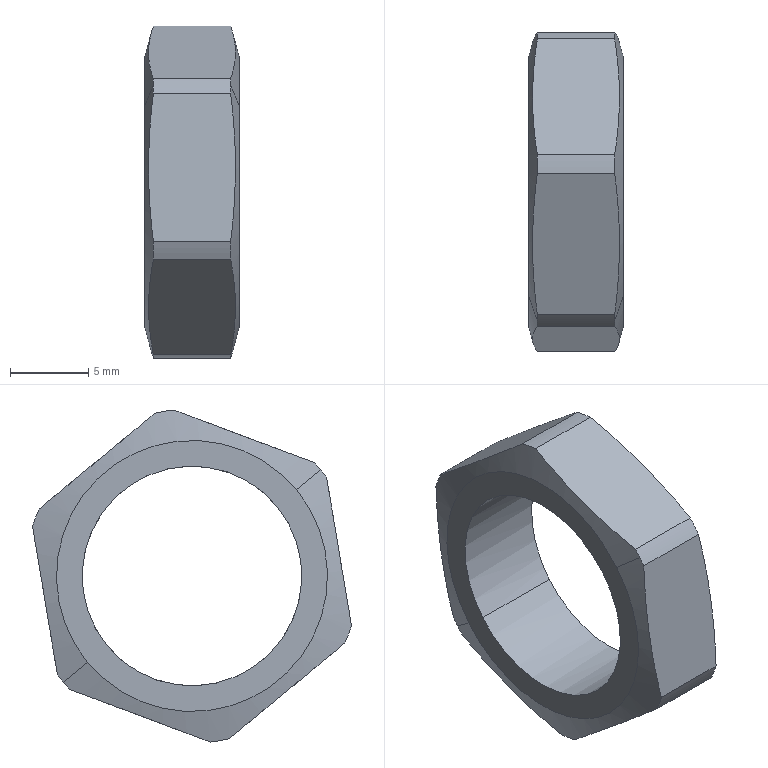Component | SolidWorks | BufferAIRTACACA_1412_2_N-1_ACA_1412_1_NT-2 | 1 solid | 21 faces | box 6 x 20.33 x 21.16 mm | volume 915 mm3 | cylinder 9 | plane 8 | cone 4 | commonest cylinder face diameters 21.289 x7 14 x2
STEP:
#1=COLOUR_RGB('',0.7922,0.8196,0.9333);
#2=FILL_AREA_STYLE_COLOUR('',#1);
#3=FILL_AREA_STYLE('',(#2));
#4=SURFACE_STYLE_FILL_AREA(#3);
#5=SURFACE_SIDE_STYLE('',(#4));
#6=SURFACE_STYLE_USAGE(.BOTH.,#5);
#7=PRESENTATION_STYLE_ASSIGNMENT((#6));
#8=CARTESIAN_POINT('',(2.52,-0.9449,-1.99));
#9=VERTEX_POINT('',#8);
#10=CARTESIAN_POINT('',(2.52,-0.5197,-2.341));
#11=VERTEX_POINT('',#10);
#12=CARTESIAN_POINT('',(2.52,-0.9449,-1.99));
#13=CARTESIAN_POINT('',(2.52,-0.9334,-1.976));
#14=CARTESIAN_POINT('',(2.52,-0.9206,-1.963));
#15=CARTESIAN_POINT('',(2.52,-0.8926,-1.94));
#16=CARTESIAN_POINT('',(2.52,-0.8776,-1.93));
#17=CARTESIAN_POINT('',(2.52,-0.8456,-1.913));
#18=CARTESIAN_POINT('',(2.52,-0.8289,-1.907));
#19=CARTESIAN_POINT('',(2.52,-0.7943,-1.896));
#20=CARTESIAN_POINT('',(2.52,-0.7766,-1.893));
#21=CARTESIAN_POINT('',(2.52,-0.7406,-1.889));
#22=CARTESIAN_POINT('',(2.52,-0.7226,-1.889));
#23=CARTESIAN_POINT('',(2.52,-0.6866,-1.893));
#24=CARTESIAN_POINT('',(2.52,-0.6689,-1.897));
#25=CARTESIAN_POINT('',(2.52,-0.6343,-1.907));
#26=CARTESIAN_POINT('',(2.52,-0.6177,-1.914));
#27=CARTESIAN_POINT('',(2.52,-0.5858,-1.931));
#28=CARTESIAN_POINT('',(2.52,-0.5709,-1.941));
#29=CARTESIAN_POINT('',(2.52,-0.543,-1.964));
#30=CARTESIAN_POINT('',(2.52,-0.5302,-1.977));
#31=CARTESIAN_POINT('',(2.52,-0.5074,-2.005));
#32=CARTESIAN_POINT('',(2.52,-0.4974,-2.02));
#33=CARTESIAN_POINT('',(2.52,-0.4804,-2.052));
#34=CARTESIAN_POINT('',(2.52,-0.4736,-2.069));
#35=CARTESIAN_POINT('',(2.52,-0.4632,-2.103));
#36=CARTESIAN_POINT('',(2.52,-0.4597,-2.121));
#37=CARTESIAN_POINT('',(2.52,-0.4562,-2.157));
#38=CARTESIAN_POINT('',(2.52,-0.4563,-2.175));
#39=CARTESIAN_POINT('',(2.52,-0.4599,-2.211));
#40=CARTESIAN_POINT('',(2.52,-0.4635,-2.229));
#41=CARTESIAN_POINT('',(2.52,-0.4741,-2.263));
#42=CARTESIAN_POINT('',(2.52,-0.481,-2.28));
#43=CARTESIAN_POINT('',(2.52,-0.4981,-2.312));
#44=CARTESIAN_POINT('',(2.52,-0.5082,-2.327));
#45=CARTESIAN_POINT('',(2.52,-0.5197,-2.341));
#46=B_SPLINE_CURVE_WITH_KNOTS('',3,(#12,#13,#14,#15,#16,#17,#18,#19,#20,#21,#22,#23,#24,#25,#26,#27,#28,#29,#30,#31,#32,#33,#34,#35,#36,#37,#38,#39,#40,#41,#42,#43,#44,#45),.UNSPECIFIED.,.F.,.F.,(4,2,2,2,2,2,2,2,2,2,2,2,2,2,2,2,4),(0.5,0.5313,0.5625,0.5938,0.625,0.6563,0.6875,0.7188,0.75,0.7813,0.8125,0.8438,0.875,0.9063,0.9375,0.9688,1.),.UNSPECIFIED.);
#47=EDGE_CURVE('',#9,#11,#46,.T.);
#48=ORIENTED_EDGE('',*,*,#47,.F.);
#49=CARTESIAN_POINT('',(2.283,-0.9449,-1.99));
#50=VERTEX_POINT('',#49);
#51=CARTESIAN_POINT('',(2.52,-0.9449,-1.99));
#52=DIRECTION('',(-1.,0.,-0.));
#53=VECTOR('',#52,39.37);
#54=LINE('',#51,#53);
#55=EDGE_CURVE('',#9,#50,#54,.T.);
#56=ORIENTED_EDGE('',*,*,#55,.T.);
#57=CARTESIAN_POINT('',(2.283,-0.5197,-2.341));
#58=VERTEX_POINT('',#57);
#59=CARTESIAN_POINT('',(2.283,-0.7323,-2.165));
#60=DIRECTION('',(-1.,0.,-0.));
#61=DIRECTION('',(0.,0.7714,-0.6363));
#62=AXIS2_PLACEMENT_3D('',#59,#60,#61);
#63=CIRCLE('',#62,0.2756);
#64=EDGE_CURVE('',#50,#58,#63,.T.);
#65=ORIENTED_EDGE('',*,*,#64,.T.);
#66=CARTESIAN_POINT('',(2.52,-0.5197,-2.341));
#67=DIRECTION('',(-1.,0.,-0.));
#68=VECTOR('',#67,39.37);
#69=LINE('',#66,#68);
#70=EDGE_CURVE('',#11,#58,#69,.T.);
#71=ORIENTED_EDGE('',*,*,#70,.F.);
#72=EDGE_LOOP('',(#48,#56,#65,#71));
#73=FACE_OUTER_BOUND('',#72,.T.);
#74=CARTESIAN_POINT('',(2.52,-0.7323,-2.165));
#75=DIRECTION('',(-1.,0.,-0.));
#76=DIRECTION('',(0.,0.7714,-0.6363));
#77=AXIS2_PLACEMENT_3D('',#74,#75,#76);
#78=CYLINDRICAL_SURFACE('',#77,0.2756);
#79=ADVANCED_FACE('',(#73),#78,.F.);
#80=CARTESIAN_POINT('',(2.499,-0.3947,-2.414));
#81=VERTEX_POINT('',#80);
#82=CARTESIAN_POINT('',(2.499,-0.409,-2.432));
#83=VERTEX_POINT('',#82);
#84=CARTESIAN_POINT('',(2.499,-0.7323,-2.165));
#85=DIRECTION('',(-1.,0.,-0.));
#86=DIRECTION('',(0.,0.7714,-0.6363));
#87=AXIS2_PLACEMENT_3D('',#84,#85,#86);
#88=CIRCLE('',#87,0.4191);
#89=EDGE_CURVE('',#81,#83,#88,.T.);
#90=ORIENTED_EDGE('',*,*,#89,.T.);
#91=CARTESIAN_POINT('',(2.305,-0.409,-2.432));
#92=VERTEX_POINT('',#91);
#93=CARTESIAN_POINT('',(2.756,-0.409,-2.432));
#94=DIRECTION('',(-1.,0.,-0.));
#95=VECTOR('',#94,39.37);
#96=LINE('',#93,#95);
#97=EDGE_CURVE('',#83,#92,#96,.T.);
#98=ORIENTED_EDGE('',*,*,#97,.T.);
#99=CARTESIAN_POINT('',(2.305,-0.3947,-2.414));
#100=VERTEX_POINT('',#99);
#101=CARTESIAN_POINT('',(2.305,-0.7323,-2.165));
#102=DIRECTION('',(1.,-0.,0.));
#103=DIRECTION('',(0.,-0.7714,0.6363));
#104=AXIS2_PLACEMENT_3D('',#101,#102,#103);
#105=CIRCLE('',#104,0.4191);
#106=EDGE_CURVE('',#92,#100,#105,.T.);
#107=ORIENTED_EDGE('',*,*,#106,.T.);
#108=CARTESIAN_POINT('',(2.756,-0.3947,-2.414));
#109=DIRECTION('',(-1.,0.,-0.));
#110=VECTOR('',#109,39.37);
#111=LINE('',#108,#110);
#112=EDGE_CURVE('',#81,#100,#111,.T.);
#113=ORIENTED_EDGE('',*,*,#112,.F.);
#114=EDGE_LOOP('',(#90,#98,#107,#113));
#115=FACE_OUTER_BOUND('',#114,.T.);
#116=CARTESIAN_POINT('',(2.756,-0.7323,-2.165));
#117=DIRECTION('',(-1.,0.,-0.));
#118=DIRECTION('',(0.,0.7714,-0.6363));
#119=AXIS2_PLACEMENT_3D('',#116,#117,#118);
#120=CYLINDRICAL_SURFACE('',#119,0.4191);
#121=ADVANCED_FACE('',(#115),#120,.T.);
#122=CARTESIAN_POINT('',(2.283,-0.47,-2.382));
#123=VERTEX_POINT('',#122);
#124=CARTESIAN_POINT('',(2.283,-0.9946,-1.949));
#125=VERTEX_POINT('',#124);
#126=CARTESIAN_POINT('',(2.283,-0.7323,-2.165));
#127=DIRECTION('',(-1.,0.,-0.));
#128=DIRECTION('',(0.,0.7714,-0.6363));
#129=AXIS2_PLACEMENT_3D('',#126,#127,#128);
#130=CIRCLE('',#129,0.34);
#131=EDGE_CURVE('',#123,#125,#130,.T.);
#132=ORIENTED_EDGE('',*,*,#131,.F.);
#133=CARTESIAN_POINT('',(2.402,-0.13,-2.662));
#134=DIRECTION('',(0.2588,0.7451,-0.6147));
#135=VECTOR('',#134,39.37);
#136=LINE('',#133,#135);
#137=EDGE_CURVE('',#123,#92,#136,.T.);
#138=ORIENTED_EDGE('',*,*,#137,.T.);
#139=CARTESIAN_POINT('',(2.305,-0.4243,-2.45));
#140=VERTEX_POINT('',#139);
#141=CARTESIAN_POINT('',(2.305,-0.7323,-2.165));
#142=DIRECTION('',(1.,-0.,0.));
#143=DIRECTION('',(0.,-0.7714,0.6363));
#144=AXIS2_PLACEMENT_3D('',#141,#142,#143);
#145=CIRCLE('',#144,0.4191);
#146=EDGE_CURVE('',#140,#92,#145,.T.);
#147=ORIENTED_EDGE('',*,*,#146,.F.);
#148=CARTESIAN_POINT('',(2.305,-0.7785,-2.582));
#149=VERTEX_POINT('',#148);
#150=CARTESIAN_POINT('',(2.305,-0.7785,-2.582));
#151=CARTESIAN_POINT('',(2.297,-0.7195,-2.56));
#152=CARTESIAN_POINT('',(2.288,-0.6014,-2.516));
#153=CARTESIAN_POINT('',(2.297,-0.4834,-2.472));
#154=CARTESIAN_POINT('',(2.305,-0.4243,-2.45));
#155=B_SPLINE_CURVE_WITH_KNOTS('',3,(#150,#151,#152,#153,#154),.UNSPECIFIED.,.F.,.F.,(4,1,4),(0.000684,0.005485,0.01029),.UNSPECIFIED.);
#156=EDGE_CURVE('',#149,#140,#155,.T.);
#157=ORIENTED_EDGE('',*,*,#156,.F.);
#158=CARTESIAN_POINT('',(2.305,-0.8245,-2.574));
#159=VERTEX_POINT('',#158);
#160=CARTESIAN_POINT('',(2.305,-0.7323,-2.165));
#161=DIRECTION('',(1.,-0.,0.));
#162=DIRECTION('',(0.,-0.7714,0.6363));
#163=AXIS2_PLACEMENT_3D('',#160,#161,#162);
#164=CIRCLE('',#163,0.4191);
#165=EDGE_CURVE('',#159,#149,#164,.T.);
#166=ORIENTED_EDGE('',*,*,#165,.F.);
#167=CARTESIAN_POINT('',(2.305,-1.116,-2.334));
#168=VERTEX_POINT('',#167);
#169=CARTESIAN_POINT('',(2.305,-1.116,-2.334));
#170=CARTESIAN_POINT('',(2.301,-1.092,-2.354));
#171=CARTESIAN_POINT('',(2.298,-1.067,-2.374));
#172=CARTESIAN_POINT('',(2.294,-1.019,-2.414));
#173=CARTESIAN_POINT('',(2.293,-0.9943,-2.434));
#174=CARTESIAN_POINT('',(2.293,-0.9214,-2.494));
#175=CARTESIAN_POINT('',(2.297,-0.8729,-2.534));
#176=CARTESIAN_POINT('',(2.305,-0.8245,-2.574));
#177=B_SPLINE_CURVE_WITH_KNOTS('',3,(#169,#170,#171,#172,#173,#174,#175,#176),.UNSPECIFIED.,.F.,.F.,(4,2,2,4),(0.01002,0.01244,0.01485,0.01969),.UNSPECIFIED.);
#178=EDGE_CURVE('',#168,#159,#177,.T.);
#179=ORIENTED_EDGE('',*,*,#178,.F.);
#180=CARTESIAN_POINT('',(2.305,-1.132,-2.29));
#181=VERTEX_POINT('',#180);
#182=CARTESIAN_POINT('',(2.305,-0.7323,-2.165));
#183=DIRECTION('',(1.,-0.,0.));
#184=DIRECTION('',(0.,-0.7714,0.6363));
#185=AXIS2_PLACEMENT_3D('',#182,#183,#184);
#186=CIRCLE('',#185,0.4191);
#187=EDGE_CURVE('',#181,#168,#186,.T.);
#188=ORIENTED_EDGE('',*,*,#187,.F.);
#189=CARTESIAN_POINT('',(2.305,-1.07,-1.917));
#190=VERTEX_POINT('',#189);
#191=CARTESIAN_POINT('',(2.305,-1.07,-1.917));
#192=CARTESIAN_POINT('',(2.297,-1.08,-1.979));
#193=CARTESIAN_POINT('',(2.288,-1.101,-2.103));
#194=CARTESIAN_POINT('',(2.297,-1.122,-2.228));
#195=CARTESIAN_POINT('',(2.305,-1.132,-2.29));
#196=B_SPLINE_CURVE_WITH_KNOTS('',3,(#191,#192,#193,#194,#195),.UNSPECIFIED.,.F.,.F.,(4,1,4),(0.000684,0.005485,0.01029),.UNSPECIFIED.);
#197=EDGE_CURVE('',#190,#181,#196,.T.);
#198=ORIENTED_EDGE('',*,*,#197,.F.);
#199=CARTESIAN_POINT('',(2.305,-1.056,-1.899));
#200=VERTEX_POINT('',#199);
#201=CARTESIAN_POINT('',(2.305,-0.7323,-2.165));
#202=DIRECTION('',(1.,-0.,0.));
#203=DIRECTION('',(0.,-0.7714,0.6363));
#204=AXIS2_PLACEMENT_3D('',#201,#202,#203);
#205=CIRCLE('',#204,0.4191);
#206=EDGE_CURVE('',#200,#190,#205,.T.);
#207=ORIENTED_EDGE('',*,*,#206,.F.);
#208=CARTESIAN_POINT('',(2.402,-1.335,-1.668));
#209=DIRECTION('',(0.2588,-0.7451,0.6147));
#210=VECTOR('',#209,39.37);
#211=LINE('',#208,#210);
#212=EDGE_CURVE('',#125,#200,#211,.T.);
#213=ORIENTED_EDGE('',*,*,#212,.F.);
#214=EDGE_LOOP('',(#132,#138,#147,#157,#166,#179,#188,#198,#207,#213));
#215=FACE_OUTER_BOUND('',#214,.T.);
#216=CARTESIAN_POINT('',(2.402,-0.7323,-2.165));
#217=DIRECTION('',(1.,-0.,0.));
#218=DIRECTION('',(0.,-0.7714,0.6363));
#219=AXIS2_PLACEMENT_3D('',#216,#217,#218);
#220=CONICAL_SURFACE('',#219,0.7808,1.309);
#221=ADVANCED_FACE('',(#215),#220,.T.);
#222=CARTESIAN_POINT('',(2.52,-0.47,-2.382));
#223=VERTEX_POINT('',#222);
#224=CARTESIAN_POINT('',(2.52,-0.9946,-1.949));
#225=VERTEX_POINT('',#224);
#226=CARTESIAN_POINT('',(2.52,-0.7323,-2.165));
#227=DIRECTION('',(-1.,0.,-0.));
#228=DIRECTION('',(0.,0.7714,-0.6363));
#229=AXIS2_PLACEMENT_3D('',#226,#227,#228);
#230=CIRCLE('',#229,0.34);
#231=EDGE_CURVE('',#223,#225,#230,.T.);
#232=ORIENTED_EDGE('',*,*,#231,.T.);
#233=CARTESIAN_POINT('',(2.499,-1.056,-1.899));
#234=VERTEX_POINT('',#233);
#235=CARTESIAN_POINT('',(2.52,-0.9946,-1.949));
#236=DIRECTION('',(-0.2588,-0.7451,0.6147));
#237=VECTOR('',#236,39.37);
#238=LINE('',#235,#237);
#239=EDGE_CURVE('',#225,#234,#238,.T.);
#240=ORIENTED_EDGE('',*,*,#239,.T.);
#241=CARTESIAN_POINT('',(2.499,-1.07,-1.917));
#242=VERTEX_POINT('',#241);
#243=CARTESIAN_POINT('',(2.499,-0.7323,-2.165));
#244=DIRECTION('',(-1.,0.,-0.));
#245=DIRECTION('',(0.,0.7714,-0.6363));
#246=AXIS2_PLACEMENT_3D('',#243,#244,#245);
#247=CIRCLE('',#246,0.4191);
#248=EDGE_CURVE('',#242,#234,#247,.T.);
#249=ORIENTED_EDGE('',*,*,#248,.F.);
#250=CARTESIAN_POINT('',(2.499,-1.132,-2.29));
#251=VERTEX_POINT('',#250);
#252=CARTESIAN_POINT('',(2.499,-1.132,-2.29));
#253=CARTESIAN_POINT('',(2.506,-1.122,-2.228));
#254=CARTESIAN_POINT('',(2.515,-1.101,-2.103));
#255=CARTESIAN_POINT('',(2.506,-1.08,-1.979));
#256=CARTESIAN_POINT('',(2.499,-1.07,-1.917));
#257=B_SPLINE_CURVE_WITH_KNOTS('',3,(#252,#253,#254,#255,#256),.UNSPECIFIED.,.F.,.F.,(4,1,4),(0.000684,0.005485,0.01029),.UNSPECIFIED.);
#258=EDGE_CURVE('',#251,#242,#257,.T.);
#259=ORIENTED_EDGE('',*,*,#258,.F.);
#260=CARTESIAN_POINT('',(2.499,-1.116,-2.334));
#261=VERTEX_POINT('',#260);
#262=CARTESIAN_POINT('',(2.499,-0.7323,-2.165));
#263=DIRECTION('',(-1.,0.,-0.));
#264=DIRECTION('',(0.,0.7714,-0.6363));
#265=AXIS2_PLACEMENT_3D('',#262,#263,#264);
#266=CIRCLE('',#265,0.4191);
#267=EDGE_CURVE('',#261,#251,#266,.T.);
#268=ORIENTED_EDGE('',*,*,#267,.F.);
#269=CARTESIAN_POINT('',(2.499,-0.8245,-2.574));
#270=VERTEX_POINT('',#269);
#271=CARTESIAN_POINT('',(2.499,-0.8245,-2.574));
#272=CARTESIAN_POINT('',(2.506,-0.8729,-2.534));
#273=CARTESIAN_POINT('',(2.511,-0.9214,-2.494));
#274=CARTESIAN_POINT('',(2.511,-0.9943,-2.434));
#275=CARTESIAN_POINT('',(2.51,-1.019,-2.414));
#276=CARTESIAN_POINT('',(2.505,-1.067,-2.374));
#277=CARTESIAN_POINT('',(2.502,-1.092,-2.354));
#278=CARTESIAN_POINT('',(2.499,-1.116,-2.334));
#279=B_SPLINE_CURVE_WITH_KNOTS('',3,(#271,#272,#273,#274,#275,#276,#277,#278),.UNSPECIFIED.,.F.,.F.,(4,2,2,4),(0.02342,0.02824,0.03065,0.03306),.UNSPECIFIED.);
#280=EDGE_CURVE('',#270,#261,#279,.T.);
#281=ORIENTED_EDGE('',*,*,#280,.F.);
#282=CARTESIAN_POINT('',(2.499,-0.7785,-2.582));
#283=VERTEX_POINT('',#282);
#284=CARTESIAN_POINT('',(2.499,-0.7323,-2.165));
#285=DIRECTION('',(-1.,0.,-0.));
#286=DIRECTION('',(0.,0.7714,-0.6363));
#287=AXIS2_PLACEMENT_3D('',#284,#285,#286);
#288=CIRCLE('',#287,0.4191);
#289=EDGE_CURVE('',#283,#270,#288,.T.);
#290=ORIENTED_EDGE('',*,*,#289,.F.);
#291=CARTESIAN_POINT('',(2.499,-0.4243,-2.45));
#292=VERTEX_POINT('',#291);
#293=CARTESIAN_POINT('',(2.499,-0.4243,-2.45));
#294=CARTESIAN_POINT('',(2.506,-0.4834,-2.472));
#295=CARTESIAN_POINT('',(2.515,-0.6014,-2.516));
#296=CARTESIAN_POINT('',(2.506,-0.7195,-2.56));
#297=CARTESIAN_POINT('',(2.499,-0.7785,-2.582));
#298=B_SPLINE_CURVE_WITH_KNOTS('',3,(#293,#294,#295,#296,#297),.UNSPECIFIED.,.F.,.F.,(4,1,4),(0.000684,0.005485,0.01029),.UNSPECIFIED.);
#299=EDGE_CURVE('',#292,#283,#298,.T.);
#300=ORIENTED_EDGE('',*,*,#299,.F.);
#301=CARTESIAN_POINT('',(2.499,-0.7323,-2.165));
#302=DIRECTION('',(-1.,0.,-0.));
#303=DIRECTION('',(0.,0.7714,-0.6363));
#304=AXIS2_PLACEMENT_3D('',#301,#302,#303);
#305=CIRCLE('',#304,0.4191);
#306=EDGE_CURVE('',#83,#292,#305,.T.);
#307=ORIENTED_EDGE('',*,*,#306,.F.);
#308=CARTESIAN_POINT('',(2.52,-0.47,-2.382));
#309=DIRECTION('',(-0.2588,0.7451,-0.6147));
#310=VECTOR('',#309,39.37);
#311=LINE('',#308,#310);
#312=EDGE_CURVE('',#223,#83,#311,.T.);
#313=ORIENTED_EDGE('',*,*,#312,.F.);
#314=EDGE_LOOP('',(#232,#240,#249,#259,#268,#281,#290,#300,#307,#313));
#315=FACE_OUTER_BOUND('',#314,.T.);
#316=CARTESIAN_POINT('',(2.52,-0.7323,-2.165));
#317=DIRECTION('',(-1.,0.,-0.));
#318=DIRECTION('',(0.,0.7714,-0.6363));
#319=AXIS2_PLACEMENT_3D('',#316,#317,#318);
#320=CONICAL_SURFACE('',#319,0.34,1.309);
#321=ADVANCED_FACE('',(#315),#320,.T.);
#322=ORIENTED_EDGE('',*,*,#239,.F.);
#323=CARTESIAN_POINT('',(2.52,-0.7323,-2.165));
#324=DIRECTION('',(-1.,0.,-0.));
#325=DIRECTION('',(0.,0.7714,-0.6363));
#326=AXIS2_PLACEMENT_3D('',#323,#324,#325);
#327=CIRCLE('',#326,0.34);
#328=EDGE_CURVE('',#225,#223,#327,.T.);
#329=ORIENTED_EDGE('',*,*,#328,.T.);
#330=ORIENTED_EDGE('',*,*,#312,.T.);
#331=ORIENTED_EDGE('',*,*,#89,.F.);
#332=CARTESIAN_POINT('',(2.499,-0.3322,-2.041));
#333=VERTEX_POINT('',#332);
#334=CARTESIAN_POINT('',(2.499,-0.3322,-2.041));
#335=CARTESIAN_POINT('',(2.506,-0.3426,-2.103));
#336=CARTESIAN_POINT('',(2.515,-0.3634,-2.227));
#337=CARTESIAN_POINT('',(2.506,-0.3843,-2.351));
#338=CARTESIAN_POINT('',(2.499,-0.3947,-2.414));
#339=B_SPLINE_CURVE_WITH_KNOTS('',3,(#334,#335,#336,#337,#338),.UNSPECIFIED.,.F.,.F.,(4,1,4),(0.000684,0.005485,0.01029),.UNSPECIFIED.);
#340=EDGE_CURVE('',#333,#81,#339,.T.);
#341=ORIENTED_EDGE('',*,*,#340,.F.);
#342=CARTESIAN_POINT('',(2.499,-0.3485,-1.997));
#343=VERTEX_POINT('',#342);
#344=CARTESIAN_POINT('',(2.499,-0.7323,-2.165));
#345=DIRECTION('',(-1.,0.,-0.));
#346=DIRECTION('',(0.,0.7714,-0.6363));
#347=AXIS2_PLACEMENT_3D('',#344,#345,#346);
#348=CIRCLE('',#347,0.4191);
#349=EDGE_CURVE('',#343,#333,#348,.T.);
#350=ORIENTED_EDGE('',*,*,#349,.F.);
#351=CARTESIAN_POINT('',(2.499,-0.6401,-1.757));
#352=VERTEX_POINT('',#351);
#353=CARTESIAN_POINT('',(2.499,-0.6401,-1.757));
#354=CARTESIAN_POINT('',(2.502,-0.6158,-1.777));
#355=CARTESIAN_POINT('',(2.505,-0.5914,-1.797));
#356=CARTESIAN_POINT('',(2.51,-0.5427,-1.837));
#357=CARTESIAN_POINT('',(2.511,-0.5183,-1.857));
#358=CARTESIAN_POINT('',(2.511,-0.4454,-1.917));
#359=CARTESIAN_POINT('',(2.506,-0.3969,-1.957));
#360=CARTESIAN_POINT('',(2.499,-0.3485,-1.997));
#361=B_SPLINE_CURVE_WITH_KNOTS('',3,(#353,#354,#355,#356,#357,#358,#359,#360),.UNSPECIFIED.,.F.,.F.,(4,2,2,4),(0.01002,0.01244,0.01485,0.01969),.UNSPECIFIED.);
#362=EDGE_CURVE('',#352,#343,#361,.T.);
#363=ORIENTED_EDGE('',*,*,#362,.F.);
#364=CARTESIAN_POINT('',(2.499,-0.6861,-1.749));
#365=VERTEX_POINT('',#364);
#366=CARTESIAN_POINT('',(2.499,-0.7323,-2.165));
#367=DIRECTION('',(-1.,0.,-0.));
#368=DIRECTION('',(0.,0.7714,-0.6363));
#369=AXIS2_PLACEMENT_3D('',#366,#367,#368);
#370=CIRCLE('',#369,0.4191);
#371=EDGE_CURVE('',#365,#352,#370,.T.);
#372=ORIENTED_EDGE('',*,*,#371,.F.);
#373=CARTESIAN_POINT('',(2.499,-1.04,-1.881));
#374=VERTEX_POINT('',#373);
#375=CARTESIAN_POINT('',(2.499,-1.04,-1.881));
#376=CARTESIAN_POINT('',(2.506,-0.9812,-1.859));
#377=CARTESIAN_POINT('',(2.515,-0.8631,-1.815));
#378=CARTESIAN_POINT('',(2.506,-0.7451,-1.771));
#379=CARTESIAN_POINT('',(2.499,-0.6861,-1.749));
#380=B_SPLINE_CURVE_WITH_KNOTS('',3,(#375,#376,#377,#378,#379),.UNSPECIFIED.,.F.,.F.,(4,1,4),(0.000684,0.005485,0.01029),.UNSPECIFIED.);
#381=EDGE_CURVE('',#374,#365,#380,.T.);
#382=ORIENTED_EDGE('',*,*,#381,.F.);
#383=CARTESIAN_POINT('',(2.499,-0.7323,-2.165));
#384=DIRECTION('',(-1.,0.,-0.));
#385=DIRECTION('',(0.,0.7714,-0.6363));
#386=AXIS2_PLACEMENT_3D('',#383,#384,#385);
#387=CIRCLE('',#386,0.4191);
#388=EDGE_CURVE('',#234,#374,#387,.T.);
#389=ORIENTED_EDGE('',*,*,#388,.F.);
#390=EDGE_LOOP('',(#322,#329,#330,#331,#341,#350,#363,#372,#382,#389));
#391=FACE_OUTER_BOUND('',#390,.T.);
#392=CARTESIAN_POINT('',(2.52,-0.7323,-2.165));
#393=DIRECTION('',(-1.,0.,-0.));
#394=DIRECTION('',(0.,0.7714,-0.6363));
#395=AXIS2_PLACEMENT_3D('',#392,#393,#394);
#396=CONICAL_SURFACE('',#395,0.34,1.309);
#397=ADVANCED_FACE('',(#391),#396,.T.);
#398=ORIENTED_EDGE('',*,*,#137,.F.);
#399=CARTESIAN_POINT('',(2.283,-0.7323,-2.165));
#400=DIRECTION('',(-1.,0.,-0.));
#401=DIRECTION('',(0.,0.7714,-0.6363));
#402=AXIS2_PLACEMENT_3D('',#399,#400,#401);
#403=CIRCLE('',#402,0.34);
#404=EDGE_CURVE('',#125,#123,#403,.T.);
#405=ORIENTED_EDGE('',*,*,#404,.F.);
#406=ORIENTED_EDGE('',*,*,#212,.T.);
#407=CARTESIAN_POINT('',(2.305,-1.04,-1.881));
#408=VERTEX_POINT('',#407);
#409=CARTESIAN_POINT('',(2.305,-0.7323,-2.165));
#410=DIRECTION('',(1.,-0.,0.));
#411=DIRECTION('',(0.,-0.7714,0.6363));
#412=AXIS2_PLACEMENT_3D('',#409,#410,#411);
#413=CIRCLE('',#412,0.4191);
#414=EDGE_CURVE('',#408,#200,#413,.T.);
#415=ORIENTED_EDGE('',*,*,#414,.F.);
#416=CARTESIAN_POINT('',(2.305,-0.6861,-1.749));
#417=VERTEX_POINT('',#416);
#418=CARTESIAN_POINT('',(2.305,-0.6861,-1.749));
#419=CARTESIAN_POINT('',(2.297,-0.7451,-1.771));
#420=CARTESIAN_POINT('',(2.288,-0.8631,-1.815));
#421=CARTESIAN_POINT('',(2.297,-0.9812,-1.859));
#422=CARTESIAN_POINT('',(2.305,-1.04,-1.881));
#423=B_SPLINE_CURVE_WITH_KNOTS('',3,(#418,#419,#420,#421,#422),.UNSPECIFIED.,.F.,.F.,(4,1,4),(0.000684,0.005485,0.01029),.UNSPECIFIED.);
#424=EDGE_CURVE('',#417,#408,#423,.T.);
#425=ORIENTED_EDGE('',*,*,#424,.F.);
#426=CARTESIAN_POINT('',(2.305,-0.6401,-1.757));
#427=VERTEX_POINT('',#426);
#428=CARTESIAN_POINT('',(2.305,-0.7323,-2.165));
#429=DIRECTION('',(1.,-0.,0.));
#430=DIRECTION('',(0.,-0.7714,0.6363));
#431=AXIS2_PLACEMENT_3D('',#428,#429,#430);
#432=CIRCLE('',#431,0.4191);
#433=EDGE_CURVE('',#427,#417,#432,.T.);
#434=ORIENTED_EDGE('',*,*,#433,.F.);
#435=CARTESIAN_POINT('',(2.305,-0.3485,-1.997));
#436=VERTEX_POINT('',#435);
#437=CARTESIAN_POINT('',(2.305,-0.3485,-1.997));
#438=CARTESIAN_POINT('',(2.297,-0.3969,-1.957));
#439=CARTESIAN_POINT('',(2.293,-0.4454,-1.917));
#440=CARTESIAN_POINT('',(2.293,-0.5183,-1.857));
#441=CARTESIAN_POINT('',(2.294,-0.5427,-1.837));
#442=CARTESIAN_POINT('',(2.298,-0.5914,-1.797));
#443=CARTESIAN_POINT('',(2.301,-0.6158,-1.777));
#444=CARTESIAN_POINT('',(2.305,-0.6401,-1.757));
#445=B_SPLINE_CURVE_WITH_KNOTS('',3,(#437,#438,#439,#440,#441,#442,#443,#444),.UNSPECIFIED.,.F.,.F.,(4,2,2,4),(0.02342,0.02824,0.03065,0.03306),.UNSPECIFIED.);
#446=EDGE_CURVE('',#436,#427,#445,.T.);
#447=ORIENTED_EDGE('',*,*,#446,.F.);
#448=CARTESIAN_POINT('',(2.305,-0.3322,-2.041));
#449=VERTEX_POINT('',#448);
#450=CARTESIAN_POINT('',(2.305,-0.7323,-2.165));
#451=DIRECTION('',(1.,-0.,0.));
#452=DIRECTION('',(0.,-0.7714,0.6363));
#453=AXIS2_PLACEMENT_3D('',#450,#451,#452);
#454=CIRCLE('',#453,0.4191);
#455=EDGE_CURVE('',#449,#436,#454,.T.);
#456=ORIENTED_EDGE('',*,*,#455,.F.);
#457=CARTESIAN_POINT('',(2.305,-0.3947,-2.414));
#458=CARTESIAN_POINT('',(2.297,-0.3843,-2.351));
#459=CARTESIAN_POINT('',(2.288,-0.3634,-2.227));
#460=CARTESIAN_POINT('',(2.297,-0.3426,-2.103));
#461=CARTESIAN_POINT('',(2.305,-0.3322,-2.041));
#462=B_SPLINE_CURVE_WITH_KNOTS('',3,(#457,#458,#459,#460,#461),.UNSPECIFIED.,.F.,.F.,(4,1,4),(0.000684,0.005485,0.01029),.UNSPECIFIED.);
#463=EDGE_CURVE('',#100,#449,#462,.T.);
#464=ORIENTED_EDGE('',*,*,#463,.F.);
#465=ORIENTED_EDGE('',*,*,#106,.F.);
#466=EDGE_LOOP('',(#398,#405,#406,#415,#425,#434,#447,#456,#464,#465));
#467=FACE_OUTER_BOUND('',#466,.T.);
#468=CARTESIAN_POINT('',(2.402,-0.7323,-2.165));
#469=DIRECTION('',(1.,-0.,0.));
#470=DIRECTION('',(0.,-0.7714,0.6363));
#471=AXIS2_PLACEMENT_3D('',#468,#469,#470);
#472=CONICAL_SURFACE('',#471,0.7808,1.309);
#473=ADVANCED_FACE('',(#467),#472,.T.);
#474=ORIENTED_EDGE('',*,*,#362,.T.);
#475=CARTESIAN_POINT('',(2.756,-0.3485,-1.997));
#476=DIRECTION('',(-1.,0.,-0.));
#477=VECTOR('',#476,39.37);
#478=LINE('',#475,#477);
#479=EDGE_CURVE('',#343,#436,#478,.T.);
#480=ORIENTED_EDGE('',*,*,#479,.T.);
#481=ORIENTED_EDGE('',*,*,#446,.T.);
#482=CARTESIAN_POINT('',(2.756,-0.6401,-1.757));
#483=DIRECTION('',(1.,-0.,0.));
#484=VECTOR('',#483,39.37);
#485=LINE('',#482,#484);
#486=EDGE_CURVE('',#427,#352,#485,.T.);
#487=ORIENTED_EDGE('',*,*,#486,.T.);
#488=EDGE_LOOP('',(#474,#480,#481,#487));
#489=FACE_OUTER_BOUND('',#488,.T.);
#490=CARTESIAN_POINT('',(2.756,-0.6609,-1.739));
#491=DIRECTION('',(0.,0.6363,0.7714));
#492=DIRECTION('',(0.,0.7714,-0.6363));
#493=AXIS2_PLACEMENT_3D('',#490,#491,#492);
#494=PLANE('',#493);
#495=ADVANCED_FACE('',(#489),#494,.T.);
#496=ORIENTED_EDGE('',*,*,#381,.T.);
#497=CARTESIAN_POINT('',(2.756,-0.6861,-1.749));
#498=DIRECTION('',(-1.,0.,-0.));
#499=VECTOR('',#498,39.37);
#500=LINE('',#497,#499);
#501=EDGE_CURVE('',#365,#417,#500,.T.);
#502=ORIENTED_EDGE('',*,*,#501,.T.);
#503=ORIENTED_EDGE('',*,*,#424,.T.);
#504=CARTESIAN_POINT('',(2.756,-1.04,-1.881));
#505=DIRECTION('',(1.,-0.,0.));
#506=VECTOR('',#505,39.37);
#507=LINE('',#504,#506);
#508=EDGE_CURVE('',#408,#374,#507,.T.);
#509=ORIENTED_EDGE('',*,*,#508,.T.);
#510=EDGE_LOOP('',(#496,#502,#503,#509));
#511=FACE_OUTER_BOUND('',#510,.T.);
#512=CARTESIAN_POINT('',(2.756,-1.065,-1.891));
#513=DIRECTION('',(-0.,-0.3499,0.9368));
#514=DIRECTION('',(0.,0.9368,0.3499));
#515=AXIS2_PLACEMENT_3D('',#512,#513,#514);
#516=PLANE('',#515);
#517=ADVANCED_FACE('',(#511),#516,.T.);
#518=ORIENTED_EDGE('',*,*,#258,.T.);
#519=CARTESIAN_POINT('',(2.756,-1.07,-1.917));
#520=DIRECTION('',(-1.,0.,-0.));
#521=VECTOR('',#520,39.37);
#522=LINE('',#519,#521);
#523=EDGE_CURVE('',#242,#190,#522,.T.);
#524=ORIENTED_EDGE('',*,*,#523,.T.);
#525=ORIENTED_EDGE('',*,*,#197,.T.);
#526=CARTESIAN_POINT('',(2.756,-1.132,-2.29));
#527=DIRECTION('',(1.,-0.,0.));
#528=VECTOR('',#527,39.37);
#529=LINE('',#526,#528);
#530=EDGE_CURVE('',#181,#251,#529,.T.);
#531=ORIENTED_EDGE('',*,*,#530,.T.);
#532=EDGE_LOOP('',(#518,#524,#525,#531));
#533=FACE_OUTER_BOUND('',#532,.T.);
#534=CARTESIAN_POINT('',(2.756,-1.137,-2.316));
#535=DIRECTION('',(-0.,-0.9862,0.1654));
#536=DIRECTION('',(0.,0.1654,0.9862));
#537=AXIS2_PLACEMENT_3D('',#534,#535,#536);
#538=PLANE('',#537);
#539=ADVANCED_FACE('',(#533),#538,.T.);
#540=ORIENTED_EDGE('',*,*,#280,.T.);
#541=CARTESIAN_POINT('',(2.756,-1.116,-2.334));
#542=DIRECTION('',(-1.,0.,-0.));
#543=VECTOR('',#542,39.37);
#544=LINE('',#541,#543);
#545=EDGE_CURVE('',#261,#168,#544,.T.);
#546=ORIENTED_EDGE('',*,*,#545,.T.);
#547=ORIENTED_EDGE('',*,*,#178,.T.);
#548=CARTESIAN_POINT('',(2.756,-0.8245,-2.574));
#549=DIRECTION('',(1.,-0.,0.));
#550=VECTOR('',#549,39.37);
#551=LINE('',#548,#550);
#552=EDGE_CURVE('',#159,#270,#551,.T.);
#553=ORIENTED_EDGE('',*,*,#552,.T.);
#554=EDGE_LOOP('',(#540,#546,#547,#553));
#555=FACE_OUTER_BOUND('',#554,.T.);
#556=CARTESIAN_POINT('',(2.756,-0.8037,-2.591));
#557=DIRECTION('',(-0.,-0.6363,-0.7714));
#558=DIRECTION('',(-0.,-0.7714,0.6363));
#559=AXIS2_PLACEMENT_3D('',#556,#557,#558);
#560=PLANE('',#559);
#561=ADVANCED_FACE('',(#555),#560,.T.);
#562=ORIENTED_EDGE('',*,*,#299,.T.);
#563=CARTESIAN_POINT('',(2.756,-0.7785,-2.582));
#564=DIRECTION('',(-1.,0.,-0.));
#565=VECTOR('',#564,39.37);
#566=LINE('',#563,#565);
#567=EDGE_CURVE('',#283,#149,#566,.T.);
#568=ORIENTED_EDGE('',*,*,#567,.T.);
#569=ORIENTED_EDGE('',*,*,#156,.T.);
#570=CARTESIAN_POINT('',(2.756,-0.4243,-2.45));
#571=DIRECTION('',(1.,-0.,0.));
#572=VECTOR('',#571,39.37);
#573=LINE('',#570,#572);
#574=EDGE_CURVE('',#140,#292,#573,.T.);
#575=ORIENTED_EDGE('',*,*,#574,.T.);
#576=EDGE_LOOP('',(#562,#568,#569,#575));
#577=FACE_OUTER_BOUND('',#576,.T.);
#578=CARTESIAN_POINT('',(2.756,-0.3991,-2.44));
#579=DIRECTION('',(0.,0.3499,-0.9368));
#580=DIRECTION('',(-0.,-0.9368,-0.3499));
#581=AXIS2_PLACEMENT_3D('',#578,#579,#580);
#582=PLANE('',#581);
#583=ADVANCED_FACE('',(#577),#582,.T.);
#584=ORIENTED_EDGE('',*,*,#340,.T.);
#585=ORIENTED_EDGE('',*,*,#112,.T.);
#586=ORIENTED_EDGE('',*,*,#463,.T.);
#587=CARTESIAN_POINT('',(2.756,-0.3322,-2.041));
#588=DIRECTION('',(1.,-0.,0.));
#589=VECTOR('',#588,39.37);
#590=LINE('',#587,#589);
#591=EDGE_CURVE('',#449,#333,#590,.T.);
#592=ORIENTED_EDGE('',*,*,#591,.T.);
#593=EDGE_LOOP('',(#584,#585,#586,#592));
#594=FACE_OUTER_BOUND('',#593,.T.);
#595=CARTESIAN_POINT('',(2.756,-0.3277,-2.014));
#596=DIRECTION('',(0.,0.9862,-0.1654));
#597=DIRECTION('',(-0.,-0.1654,-0.9862));
#598=AXIS2_PLACEMENT_3D('',#595,#596,#597);
#599=PLANE('',#598);
#600=ADVANCED_FACE('',(#594),#599,.T.);
#601=ORIENTED_EDGE('',*,*,#231,.F.);
#602=ORIENTED_EDGE('',*,*,#328,.F.);
#603=EDGE_LOOP('',(#601,#602));
#604=FACE_OUTER_BOUND('',#603,.T.);
#605=CARTESIAN_POINT('',(2.52,-0.5197,-2.341));
#606=CARTESIAN_POINT('',(2.52,-0.5312,-2.355));
#607=CARTESIAN_POINT('',(2.52,-0.544,-2.367));
#608=CARTESIAN_POINT('',(2.52,-0.572,-2.39));
#609=CARTESIAN_POINT('',(2.52,-0.587,-2.4));
#610=CARTESIAN_POINT('',(2.52,-0.619,-2.417));
#611=CARTESIAN_POINT('',(2.52,-0.6356,-2.424));
#612=CARTESIAN_POINT('',(2.52,-0.6703,-2.434));
#613=CARTESIAN_POINT('',(2.52,-0.688,-2.438));
#614=CARTESIAN_POINT('',(2.52,-0.724,-2.441));
#615=CARTESIAN_POINT('',(2.52,-0.742,-2.441));
#616=CARTESIAN_POINT('',(2.52,-0.778,-2.438));
#617=CARTESIAN_POINT('',(2.52,-0.7957,-2.434));
#618=CARTESIAN_POINT('',(2.52,-0.8302,-2.424));
#619=CARTESIAN_POINT('',(2.52,-0.8469,-2.417));
#620=CARTESIAN_POINT('',(2.52,-0.8787,-2.4));
#621=CARTESIAN_POINT('',(2.52,-0.8937,-2.389));
#622=CARTESIAN_POINT('',(2.52,-0.9216,-2.366));
#623=CARTESIAN_POINT('',(2.52,-0.9343,-2.354));
#624=CARTESIAN_POINT('',(2.52,-0.9572,-2.326));
#625=CARTESIAN_POINT('',(2.52,-0.9672,-2.311));
#626=CARTESIAN_POINT('',(2.52,-0.9841,-2.279));
#627=CARTESIAN_POINT('',(2.52,-0.991,-2.262));
#628=CARTESIAN_POINT('',(2.52,-1.001,-2.227));
#629=CARTESIAN_POINT('',(2.52,-1.005,-2.21));
#630=CARTESIAN_POINT('',(2.52,-1.008,-2.174));
#631=CARTESIAN_POINT('',(2.52,-1.008,-2.156));
#632=CARTESIAN_POINT('',(2.52,-1.005,-2.12));
#633=CARTESIAN_POINT('',(2.52,-1.001,-2.102));
#634=CARTESIAN_POINT('',(2.52,-0.9905,-2.067));
#635=CARTESIAN_POINT('',(2.52,-0.9836,-2.051));
#636=CARTESIAN_POINT('',(2.52,-0.9664,-2.019));
#637=CARTESIAN_POINT('',(2.52,-0.9564,-2.004));
#638=CARTESIAN_POINT('',(2.52,-0.9449,-1.99));
#639=B_SPLINE_CURVE_WITH_KNOTS('',3,(#605,#606,#607,#608,#609,#610,#611,#612,#613,#614,#615,#616,#617,#618,#619,#620,#621,#622,#623,#624,#625,#626,#627,#628,#629,#630,#631,#632,#633,#634,#635,#636,#637,#638),.UNSPECIFIED.,.F.,.F.,(4,2,2,2,2,2,2,2,2,2,2,2,2,2,2,2,4),(0.,0.03125,0.0625,0.09375,0.125,0.1562,0.1875,0.2188,0.25,0.2812,0.3125,0.3438,0.375,0.4062,0.4375,0.4688,0.5),.UNSPECIFIED.);
#640=EDGE_CURVE('',#11,#9,#639,.T.);
#641=ORIENTED_EDGE('',*,*,#640,.T.);
#642=ORIENTED_EDGE('',*,*,#47,.T.);
#643=EDGE_LOOP('',(#641,#642));
#644=FACE_BOUND('',#643,.T.);
#645=CARTESIAN_POINT('',(2.52,-0.9077,-2.378));
#646=DIRECTION('',(-1.,0.,-0.));
#647=DIRECTION('',(0.,0.7714,-0.6363));
#648=AXIS2_PLACEMENT_3D('',#645,#646,#647);
#649=PLANE('',#648);
#650=ADVANCED_FACE('',(#604,#644),#649,.F.);
#651=CARTESIAN_POINT('',(2.283,-0.7323,-2.165));
#652=DIRECTION('',(-1.,0.,-0.));
#653=DIRECTION('',(0.,0.7714,-0.6363));
#654=AXIS2_PLACEMENT_3D('',#651,#652,#653);
#655=CIRCLE('',#654,0.2756);
#656=EDGE_CURVE('',#58,#50,#655,.T.);
#657=ORIENTED_EDGE('',*,*,#656,.F.);
#658=ORIENTED_EDGE('',*,*,#64,.F.);
#659=EDGE_LOOP('',(#657,#658));
#660=FACE_BOUND('',#659,.T.);
#661=ORIENTED_EDGE('',*,*,#404,.T.);
#662=ORIENTED_EDGE('',*,*,#131,.T.);
#663=EDGE_LOOP('',(#661,#662));
#664=FACE_OUTER_BOUND('',#663,.T.);
#665=CARTESIAN_POINT('',(2.283,-0.9486,-2.428));
#666=DIRECTION('',(1.,-0.,0.));
#667=DIRECTION('',(-0.,-0.7714,0.6363));
#668=AXIS2_PLACEMENT_3D('',#665,#666,#667);
#669=PLANE('',#668);
#670=ADVANCED_FACE('',(#660,#664),#669,.F.);
#671=ORIENTED_EDGE('',*,*,#349,.T.);
#672=ORIENTED_EDGE('',*,*,#591,.F.);
#673=ORIENTED_EDGE('',*,*,#455,.T.);
#674=ORIENTED_EDGE('',*,*,#479,.F.);
#675=EDGE_LOOP('',(#671,#672,#673,#674));
#676=FACE_OUTER_BOUND('',#675,.T.);
#677=CARTESIAN_POINT('',(2.756,-0.7323,-2.165));
#678=DIRECTION('',(-1.,0.,-0.));
#679=DIRECTION('',(0.,0.7714,-0.6363));
#680=AXIS2_PLACEMENT_3D('',#677,#678,#679);
#681=CYLINDRICAL_SURFACE('',#680,0.4191);
#682=ADVANCED_FACE('',(#676),#681,.T.);
#683=ORIENTED_EDGE('',*,*,#97,.F.);
#684=ORIENTED_EDGE('',*,*,#306,.T.);
#685=ORIENTED_EDGE('',*,*,#574,.F.);
#686=ORIENTED_EDGE('',*,*,#146,.T.);
#687=EDGE_LOOP('',(#683,#684,#685,#686));
#688=FACE_OUTER_BOUND('',#687,.T.);
#689=CARTESIAN_POINT('',(2.756,-0.7323,-2.165));
#690=DIRECTION('',(-1.,0.,-0.));
#691=DIRECTION('',(0.,0.7714,-0.6363));
#692=AXIS2_PLACEMENT_3D('',#689,#690,#691);
#693=CYLINDRICAL_SURFACE('',#692,0.4191);
#694=ADVANCED_FACE('',(#688),#693,.T.);
#695=ORIENTED_EDGE('',*,*,#165,.T.);
#696=ORIENTED_EDGE('',*,*,#567,.F.);
#697=ORIENTED_EDGE('',*,*,#289,.T.);
#698=ORIENTED_EDGE('',*,*,#552,.F.);
#699=EDGE_LOOP('',(#695,#696,#697,#698));
#700=FACE_OUTER_BOUND('',#699,.T.);
#701=CARTESIAN_POINT('',(2.756,-0.7323,-2.165));
#702=DIRECTION('',(-1.,0.,-0.));
#703=DIRECTION('',(0.,0.7714,-0.6363));
#704=AXIS2_PLACEMENT_3D('',#701,#702,#703);
#705=CYLINDRICAL_SURFACE('',#704,0.4191);
#706=ADVANCED_FACE('',(#700),#705,.T.);
#707=ORIENTED_EDGE('',*,*,#187,.T.);
#708=ORIENTED_EDGE('',*,*,#545,.F.);
#709=ORIENTED_EDGE('',*,*,#267,.T.);
#710=ORIENTED_EDGE('',*,*,#530,.F.);
#711=EDGE_LOOP('',(#707,#708,#709,#710));
#712=FACE_OUTER_BOUND('',#711,.T.);
#713=CARTESIAN_POINT('',(2.756,-0.7323,-2.165));
#714=DIRECTION('',(-1.,0.,-0.));
#715=DIRECTION('',(0.,0.7714,-0.6363));
#716=AXIS2_PLACEMENT_3D('',#713,#714,#715);
#717=CYLINDRICAL_SURFACE('',#716,0.4191);
#718=ADVANCED_FACE('',(#712),#717,.T.);
#719=ORIENTED_EDGE('',*,*,#414,.T.);
#720=ORIENTED_EDGE('',*,*,#206,.T.);
#721=ORIENTED_EDGE('',*,*,#523,.F.);
#722=ORIENTED_EDGE('',*,*,#248,.T.);
#723=ORIENTED_EDGE('',*,*,#388,.T.);
#724=ORIENTED_EDGE('',*,*,#508,.F.);
#725=EDGE_LOOP('',(#719,#720,#721,#722,#723,#724));
#726=FACE_OUTER_BOUND('',#725,.T.);
#727=CARTESIAN_POINT('',(2.756,-0.7323,-2.165));
#728=DIRECTION('',(-1.,0.,-0.));
#729=DIRECTION('',(0.,0.7714,-0.6363));
#730=AXIS2_PLACEMENT_3D('',#727,#728,#729);
#731=CYLINDRICAL_SURFACE('',#730,0.4191);
#732=ADVANCED_FACE('',(#726),#731,.T.);
#733=ORIENTED_EDGE('',*,*,#433,.T.);
#734=ORIENTED_EDGE('',*,*,#501,.F.);
#735=ORIENTED_EDGE('',*,*,#371,.T.);
#736=ORIENTED_EDGE('',*,*,#486,.F.);
#737=EDGE_LOOP('',(#733,#734,#735,#736));
#738=FACE_OUTER_BOUND('',#737,.T.);
#739=CARTESIAN_POINT('',(2.756,-0.7323,-2.165));
#740=DIRECTION('',(-1.,0.,-0.));
#741=DIRECTION('',(0.,0.7714,-0.6363));
#742=AXIS2_PLACEMENT_3D('',#739,#740,#741);
#743=CYLINDRICAL_SURFACE('',#742,0.4191);
#744=ADVANCED_FACE('',(#738),#743,.T.);
#745=ORIENTED_EDGE('',*,*,#55,.F.);
#746=ORIENTED_EDGE('',*,*,#640,.F.);
#747=ORIENTED_EDGE('',*,*,#70,.T.);
#748=ORIENTED_EDGE('',*,*,#656,.T.);
#749=EDGE_LOOP('',(#745,#746,#747,#748));
#750=FACE_OUTER_BOUND('',#749,.T.);
#751=CARTESIAN_POINT('',(2.52,-0.7323,-2.165));
#752=DIRECTION('',(-1.,0.,-0.));
#753=DIRECTION('',(0.,0.7714,-0.6363));
#754=AXIS2_PLACEMENT_3D('',#751,#752,#753);
#755=CYLINDRICAL_SURFACE('',#754,0.2756);
#756=ADVANCED_FACE('',(#750),#755,.F.);
#757=CLOSED_SHELL('',(#79,#121,#221,#321,#397,#473,#495,#517,#539,#561,#583,#600,#650,#670,#682,#694,#706,#718,#732,#744,#756));
#758=MANIFOLD_SOLID_BREP('',#757);
#759=STYLED_ITEM('',(#7),#758);
#760=(LENGTH_UNIT()NAMED_UNIT(*)SI_UNIT($,.METRE.));
#761=LENGTH_MEASURE_WITH_UNIT(LENGTH_MEASURE(0.0254),#760);
#762=DIMENSIONAL_EXPONENTS(1.,0.,0.,0.,0.,0.,0.);
#763=(CONVERSION_BASED_UNIT('',#761)LENGTH_UNIT()NAMED_UNIT(#762));
#764=UNCERTAINTY_MEASURE_WITH_UNIT(LENGTH_MEASURE(0.00001),#763,'','');
#765=(NAMED_UNIT(*)PLANE_ANGLE_UNIT()SI_UNIT($,.RADIAN.));
#766=(NAMED_UNIT(*)SI_UNIT($,.STERADIAN.)SOLID_ANGLE_UNIT());
#767=(GEOMETRIC_REPRESENTATION_CONTEXT(3)GLOBAL_UNCERTAINTY_ASSIGNED_CONTEXT((#764))GLOBAL_UNIT_ASSIGNED_CONTEXT((#763,#765,#766))REPRESENTATION_CONTEXT('',''));
#768=MECHANICAL_DESIGN_GEOMETRIC_PRESENTATION_REPRESENTATION('',(#759),#767);
#769=CARTESIAN_POINT('',(0.,0.,0.));
#770=DIRECTION('',(0.,0.,1.));
#771=DIRECTION('',(1.,0.,0.));
#772=AXIS2_PLACEMENT_3D('',#769,#770,#771);
#773=(LENGTH_UNIT()NAMED_UNIT(*)SI_UNIT($,.METRE.));
#774=LENGTH_MEASURE_WITH_UNIT(LENGTH_MEASURE(0.0254),#773);
#775=DIMENSIONAL_EXPONENTS(1.,0.,0.,0.,0.,0.,0.);
#776=(CONVERSION_BASED_UNIT('',#774)LENGTH_UNIT()NAMED_UNIT(#775));
#777=UNCERTAINTY_MEASURE_WITH_UNIT(LENGTH_MEASURE(0.00001),#776,'','');
#778=(NAMED_UNIT(*)PLANE_ANGLE_UNIT()SI_UNIT($,.RADIAN.));
#779=(NAMED_UNIT(*)SI_UNIT($,.STERADIAN.)SOLID_ANGLE_UNIT());
#780=(GEOMETRIC_REPRESENTATION_CONTEXT(3)GLOBAL_UNCERTAINTY_ASSIGNED_CONTEXT((#777))GLOBAL_UNIT_ASSIGNED_CONTEXT((#776,#778,#779))REPRESENTATION_CONTEXT('',''));
#781=ADVANCED_BREP_SHAPE_REPRESENTATION('',(#758,#772),#780);
#782=PRESENTATION_LAYER_ASSIGNMENT('','',(#759));